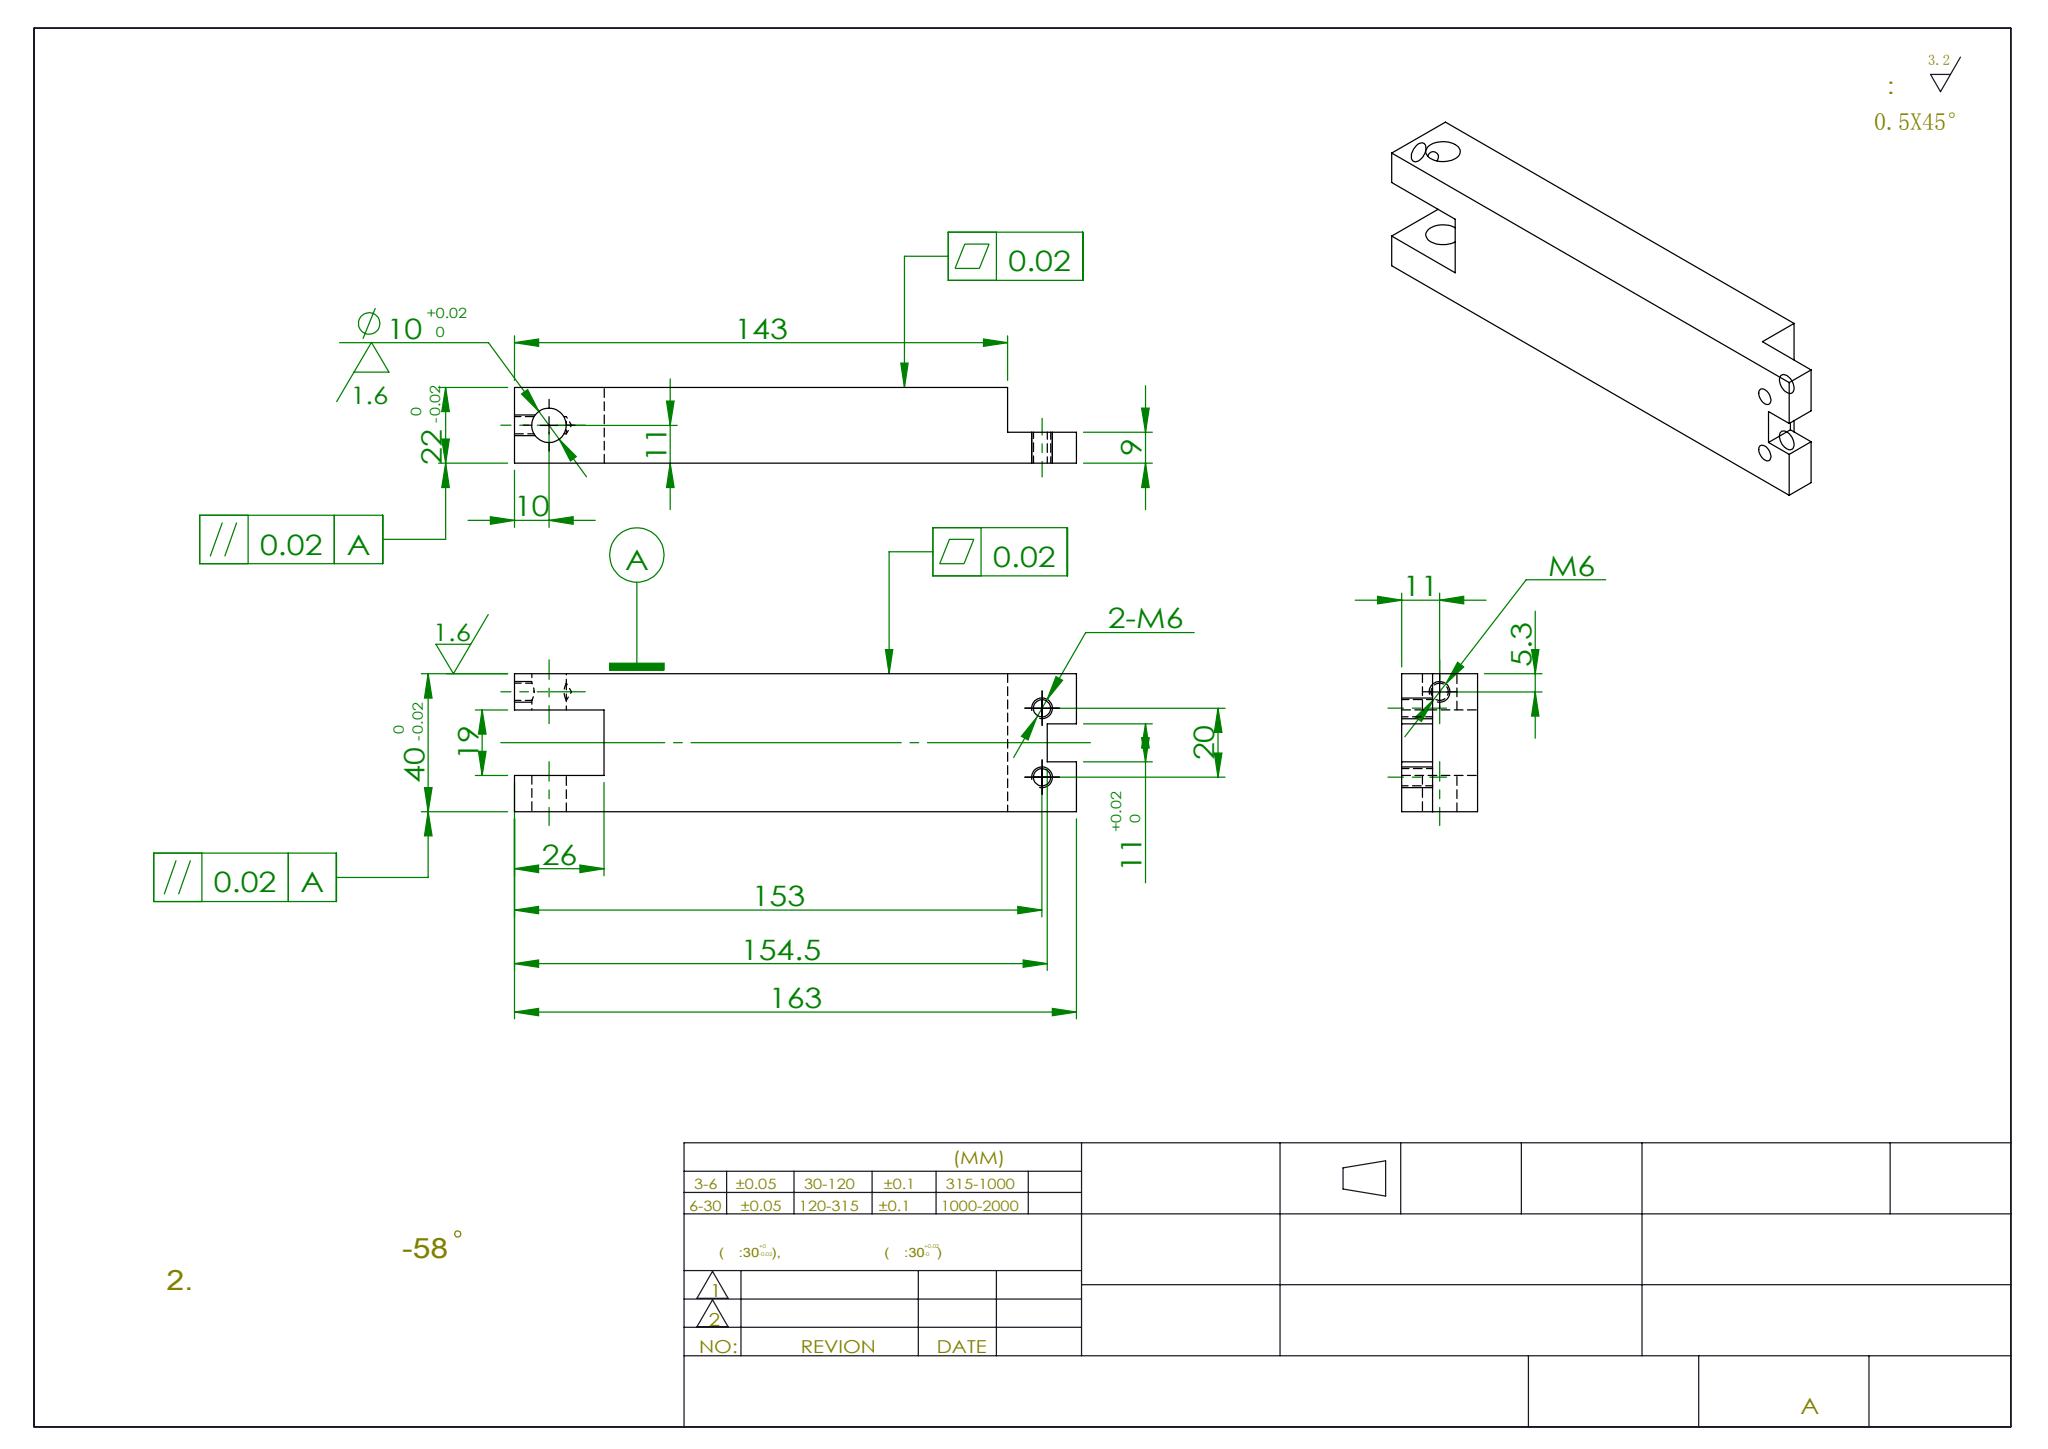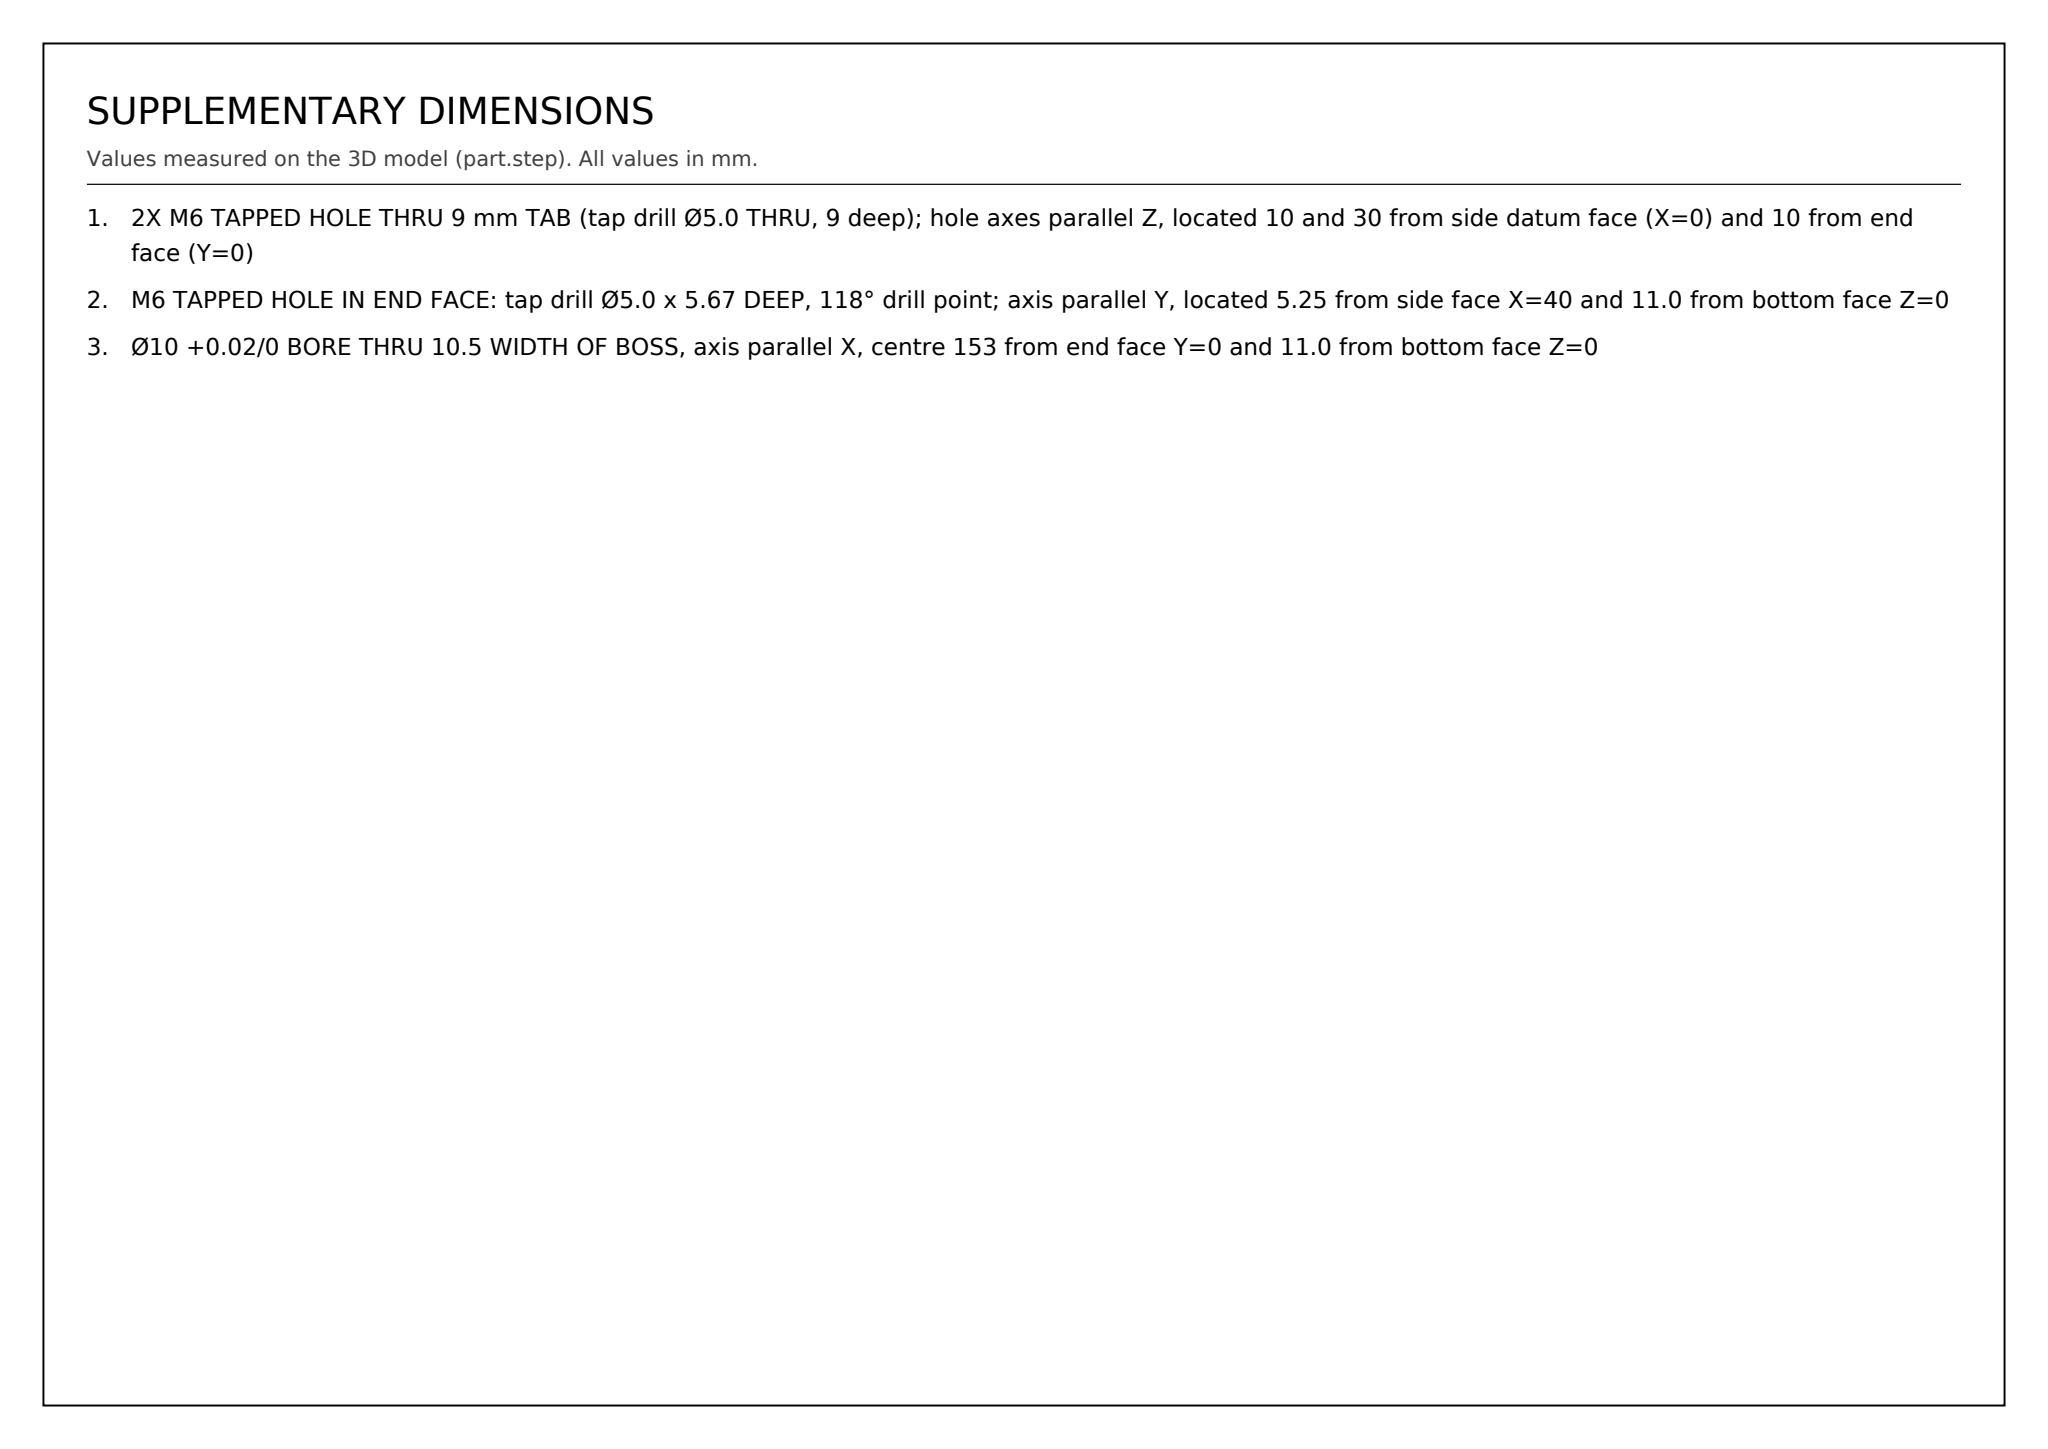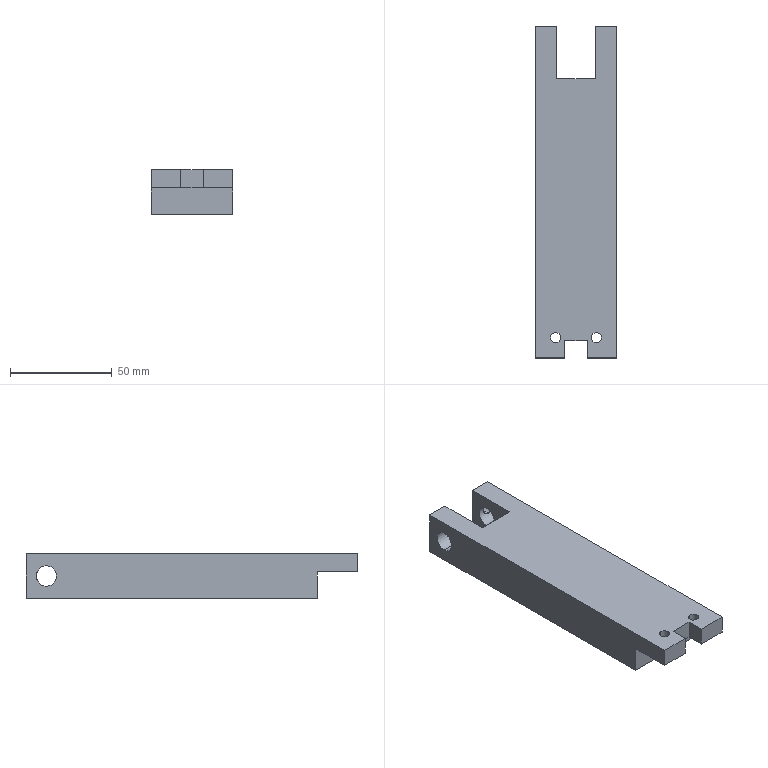Part | SolidWorks | mm | 1 solid | 31 faces | box 40 x 163 x 22 mm | volume 119213 mm3 | plane 16 | cylinder 13 | cone 2 | commonest cylinder face diameters 5 x9 10 x4
Drawing notes:
2X M6 TAPPED HOLE THRU 9 mm TAB (tap drill Ø5.0 THRU, 9 deep); hole axes parallel Z, located 10 and 30 from side datum face (X=0) and 10 from end face (Y=0) | from the solid: cylinders [5.0,"z",[10.0,10.0,null],9.0] and [5.0,"z",[30.0,10.0,null],9.0]; planes z=13.0 and z=22.0 (9 mm tab)
M6 TAPPED HOLE IN END FACE: tap drill Ø5.0 x 5.67 DEEP, 118° drill point; axis parallel Y, located 5.25 from side face X=40 and 11.0 from bottom face Z=0 | from the solid: cylinders [5.0,"y",[34.75,null,11.0],5.67] and [...,0.67]; cones [118.0,5.0]; bbox_xyz 40x163x22
Ø10 +0.02/0 BORE THRU 10.5 WIDTH OF BOSS, axis parallel X, centre 153 from end face Y=0 and 11.0 from bottom face Z=0 | from the solid: cylinder [10.0,"x",[null,153.0,11.0],10.5]; planes x=0.0 and x=10.5
build123d program:
from build123d import *

# Parameters (mm, degrees)
EXTRUDE1_DEPTH        = 20
SKETCH2_R             = 5
CUT_EXTRUDE1_DEPTH    = 170.272
SKETCH3_W             = 19
SKETCH3_H             = 26
CUT_EXTRUDE2_DEPTH    = 166.689
M6_TAPPED_HOLE1_D     = 5
M6_TAPPED_HOLE1_DEPTH = 15
M6_TAPPED_HOLE1_TIP   = 1.502
SKETCH6_W             = 11
SKETCH6_H             = 8.5
CUT_EXTRUDE3_DEPTH    = 165.736
M6_TAPPED_HOLE2_D     = 5


with BuildPart() as part:
    # Sketch1 → Extrude1 (new, symmetric)
    with BuildSketch(Plane(origin=(0, 0, 0), x_dir=(0, 0, -1), z_dir=(1, 0, 0))):
        Polygon((0, 0), (9, 0), (9, 20), (22, 20), (22, 163), (0, 163), align=None)
    extrude(amount=EXTRUDE1_DEPTH, both=True)

    # Sketch2 → Cut-Extrude1 (cut, through all)
    with BuildSketch(Plane(origin=(20, 0, 0), x_dir=(0, 0, -1), z_dir=(1, 0, 0))):
        with Locations((11, 153)):
            Circle(SKETCH2_R)
    extrude(amount=-CUT_EXTRUDE1_DEPTH, mode=Mode.SUBTRACT)

    # Sketch3 → Cut-Extrude2 (cut, through all)
    with BuildSketch(Plane(origin=(0, 0, -22), x_dir=(-1, 0, 0), z_dir=(0, 0, -1))):
        with Locations((0, 150)):
            Rectangle(SKETCH3_W, SKETCH3_H)
    extrude(amount=-CUT_EXTRUDE2_DEPTH, mode=Mode.SUBTRACT)

    # M6 Tapped Hole1
    with Locations(Plane(origin=(0, 163, 0), x_dir=(-1, 0, 0), z_dir=(0, 1, 0))):
        with Locations((-14.75, -11)):
            Hole(M6_TAPPED_HOLE1_D / 2, depth=M6_TAPPED_HOLE1_DEPTH)
            with Locations((0, 0, -(M6_TAPPED_HOLE1_DEPTH + M6_TAPPED_HOLE1_TIP / 2))):  # 118° drill point
                Cone(0, M6_TAPPED_HOLE1_D / 2, M6_TAPPED_HOLE1_TIP, mode=Mode.SUBTRACT)

    # Sketch6 → Cut-Extrude3 (cut, through all)
    with BuildSketch(Plane(origin=(0, 0, -9), x_dir=(-1, 0, 0), z_dir=(0, 0, -1))):
        with Locations((0, 4.25)):
            Rectangle(SKETCH6_W, SKETCH6_H)
    extrude(amount=-CUT_EXTRUDE3_DEPTH, mode=Mode.SUBTRACT)

    # M6 Tapped Hole2 (through all)
    with Locations(Plane(origin=(0, 0, -9), x_dir=(-1, 0, 0), z_dir=(0, 0, -1))):
        with Locations((-10, 10), (10, 10)):
            Hole(M6_TAPPED_HOLE2_D / 2)


solid = part.part